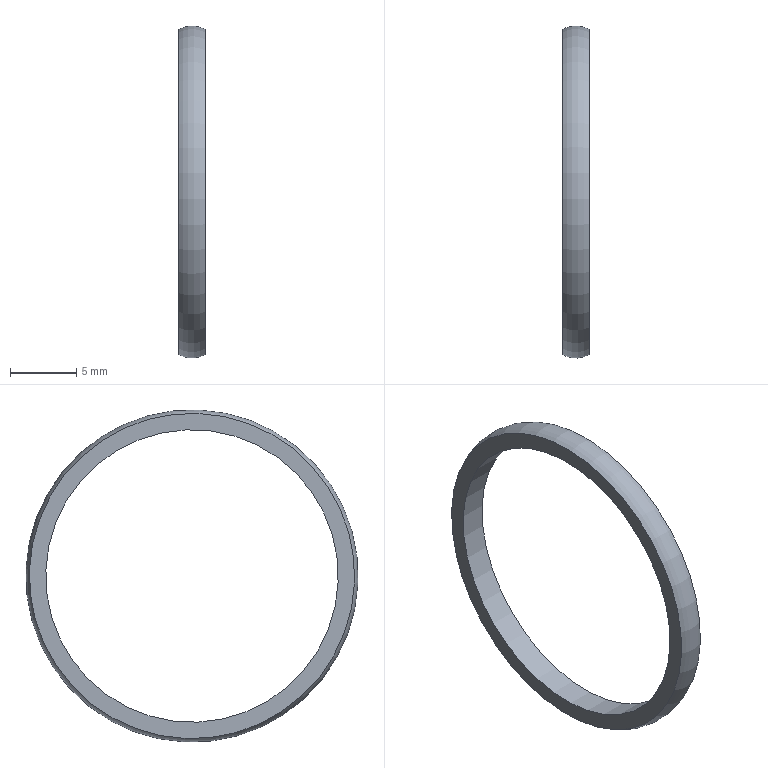Component | NX | PISTON_RING_2 | 1 solid | 4 faces | box 2 x 25 x 25 mm | volume 208 mm3 | plane 2 | torus 1 | cylinder 1 | commonest cylinder face diameters 22 x1
STEP:
#1=CARTESIAN_POINT('',(0.,0.,0.));
#2=DIRECTION('',(0.,0.,1.));
#3=DIRECTION('',(1.,0.,0.));
#4=AXIS2_PLACEMENT_3D('',#1,#2,#3);
#5=CARTESIAN_POINT('',(415.974,77.279,110.474));
#6=VERTEX_POINT('',#5);
#7=CARTESIAN_POINT('',(415.974,89.5,111.));
#8=DIRECTION('',(-1.,0.,0.));
#9=DIRECTION('',(0.,-0.9991,-0.04303));
#10=AXIS2_PLACEMENT_3D('',#7,#8,#9);
#11=CIRCLE('',#10,12.232);
#12=CARTESIAN_POINT('',(415.974,89.973,100.01));
#13=DIRECTION('',(-1.,0.,0.));
#14=DIRECTION('',(0.,-0.9991,-0.04303));
#15=AXIS2_PLACEMENT_3D('',#12,#13,#14);
#16=PLANE('',#15);
#17=CARTESIAN_POINT('',(0.,11.));
#18=DIRECTION('',(1.,-0.));
#19=AXIS2_PLACEMENT_2D('',#17,#18);
#20=CIRCLE('',#19,12.232);
#21=(GEOMETRIC_REPRESENTATION_CONTEXT(2)PARAMETRIC_REPRESENTATION_CONTEXT()REPRESENTATION_CONTEXT('',''));
#22=DEFINITIONAL_REPRESENTATION('',(#20),#21);
#23=PCURVE('',#16,#22);
#24=CARTESIAN_POINT('',(416.974,89.5,111.));
#25=DIRECTION('',(-1.,0.,0.));
#26=DIRECTION('',(0.,-0.9991,-0.04303));
#27=AXIS2_PLACEMENT_3D('',#24,#25,#26);
#28=TOROIDAL_SURFACE('',#27,10.5,2.);
#29=CARTESIAN_POINT('',(0.,6.807));
#30=DIRECTION('',(1.,0.));
#31=VECTOR('',#30,1.);
#32=LINE('',#29,#31);
#33=(GEOMETRIC_REPRESENTATION_CONTEXT(2)PARAMETRIC_REPRESENTATION_CONTEXT()REPRESENTATION_CONTEXT('',''));
#34=DEFINITIONAL_REPRESENTATION('',(#32),#33);
#35=PCURVE('',#28,#34);
#36=SURFACE_CURVE('',#11,(#23,#35),.PCURVE_S1.);
#37=EDGE_CURVE('',#6,#6,#36,.T.);
#38=ORIENTED_EDGE('',*,*,#37,.T.);
#39=EDGE_LOOP('',(#38));
#40=FACE_BOUND('',#39,.T.);
#41=CARTESIAN_POINT('',(415.974,78.51,110.527));
#42=VERTEX_POINT('',#41);
#43=CARTESIAN_POINT('',(415.974,89.5,111.));
#44=DIRECTION('',(-1.,0.,0.));
#45=DIRECTION('',(0.,-0.9991,-0.04303));
#46=AXIS2_PLACEMENT_3D('',#43,#44,#45);
#47=CIRCLE('',#46,11.);
#48=CARTESIAN_POINT('',(0.,11.));
#49=DIRECTION('',(1.,-0.));
#50=AXIS2_PLACEMENT_2D('',#48,#49);
#51=CIRCLE('',#50,11.);
#52=(GEOMETRIC_REPRESENTATION_CONTEXT(2)PARAMETRIC_REPRESENTATION_CONTEXT()REPRESENTATION_CONTEXT('',''));
#53=DEFINITIONAL_REPRESENTATION('',(#51),#52);
#54=PCURVE('',#16,#53);
#55=CARTESIAN_POINT('',(415.974,89.5,111.));
#56=DIRECTION('',(-1.,0.,0.));
#57=DIRECTION('',(0.,-0.9991,-0.04303));
#58=AXIS2_PLACEMENT_3D('',#55,#56,#57);
#59=CYLINDRICAL_SURFACE('',#58,11.);
#60=CARTESIAN_POINT('',(0.,0.));
#61=DIRECTION('',(1.,0.));
#62=VECTOR('',#61,1.);
#63=LINE('',#60,#62);
#64=(GEOMETRIC_REPRESENTATION_CONTEXT(2)PARAMETRIC_REPRESENTATION_CONTEXT()REPRESENTATION_CONTEXT('',''));
#65=DEFINITIONAL_REPRESENTATION('',(#63),#64);
#66=PCURVE('',#59,#65);
#67=SURFACE_CURVE('',#47,(#54,#66),.PCURVE_S1.);
#68=EDGE_CURVE('',#42,#42,#67,.T.);
#69=ORIENTED_EDGE('',*,*,#68,.F.);
#70=EDGE_LOOP('',(#69));
#71=FACE_BOUND('',#70,.T.);
#72=ADVANCED_FACE('',(#40,#71),#16,.T.);
#73=CARTESIAN_POINT('',(417.974,77.279,110.474));
#74=VERTEX_POINT('',#73);
#75=CARTESIAN_POINT('',(417.974,89.5,111.));
#76=DIRECTION('',(-1.,0.,0.));
#77=DIRECTION('',(0.,-0.9991,-0.04303));
#78=AXIS2_PLACEMENT_3D('',#75,#76,#77);
#79=CIRCLE('',#78,12.232);
#80=CARTESIAN_POINT('',(0.,5.76));
#81=DIRECTION('',(1.,0.));
#82=VECTOR('',#81,1.);
#83=LINE('',#80,#82);
#84=(GEOMETRIC_REPRESENTATION_CONTEXT(2)PARAMETRIC_REPRESENTATION_CONTEXT()REPRESENTATION_CONTEXT('',''));
#85=DEFINITIONAL_REPRESENTATION('',(#83),#84);
#86=PCURVE('',#28,#85);
#87=CARTESIAN_POINT('',(417.974,90.026,98.779));
#88=DIRECTION('',(1.,0.,0.));
#89=DIRECTION('',(0.,0.9991,0.04303));
#90=AXIS2_PLACEMENT_3D('',#87,#88,#89);
#91=PLANE('',#90);
#92=CARTESIAN_POINT('',(-12.232,12.232));
#93=CARTESIAN_POINT('',(-12.232,33.419));
#94=CARTESIAN_POINT('',(6.116,22.825));
#95=CARTESIAN_POINT('',(24.464,12.232));
#96=CARTESIAN_POINT('',(6.116,1.639));
#97=CARTESIAN_POINT('',(-12.232,-8.954));
#98=CARTESIAN_POINT('',(-12.232,12.232));
#99=(BOUNDED_CURVE()B_SPLINE_CURVE(2,(#92,#93,#94,#95,#96,#97,#98),.UNSPECIFIED.,.T.,.F.)B_SPLINE_CURVE_WITH_KNOTS((1,2,2,2,2,1),(-2.094,0.,2.094,4.189,6.283,8.378),.UNSPECIFIED.)CURVE()GEOMETRIC_REPRESENTATION_ITEM()RATIONAL_B_SPLINE_CURVE((1.,0.5,1.,0.5,1.,0.5,1.))REPRESENTATION_ITEM(''));
#100=(GEOMETRIC_REPRESENTATION_CONTEXT(2)PARAMETRIC_REPRESENTATION_CONTEXT()REPRESENTATION_CONTEXT('',''));
#101=DEFINITIONAL_REPRESENTATION('',(#99),#100);
#102=PCURVE('',#91,#101);
#103=SURFACE_CURVE('',#79,(#86,#102),.PCURVE_S1.);
#104=EDGE_CURVE('',#74,#74,#103,.T.);
#105=ORIENTED_EDGE('',*,*,#104,.T.);
#106=CARTESIAN_POINT('',(417.974,77.279,110.474));
#107=CARTESIAN_POINT('',(417.611,77.07,110.465));
#108=CARTESIAN_POINT('',(417.193,76.956,110.46));
#109=CARTESIAN_POINT('',(416.754,76.956,110.46));
#110=CARTESIAN_POINT('',(416.336,77.07,110.465));
#111=CARTESIAN_POINT('',(415.974,77.279,110.474));
#112=B_SPLINE_CURVE_WITH_KNOTS('',5,(#106,#107,#108,#109,#110,#111),.UNSPECIFIED.,.F.,.F.,(6,6),(5.76,6.807),.PIECEWISE_BEZIER_KNOTS.);
#113=CARTESIAN_POINT('',(6.283,0.));
#114=DIRECTION('',(0.,1.));
#115=VECTOR('',#114,1.);
#116=LINE('',#113,#115);
#117=(GEOMETRIC_REPRESENTATION_CONTEXT(2)PARAMETRIC_REPRESENTATION_CONTEXT()REPRESENTATION_CONTEXT('',''));
#118=DEFINITIONAL_REPRESENTATION('',(#116),#117);
#119=PCURVE('',#28,#118);
#120=CARTESIAN_POINT('',(0.,0.));
#121=DIRECTION('',(0.,1.));
#122=VECTOR('',#121,1.);
#123=LINE('',#120,#122);
#124=(GEOMETRIC_REPRESENTATION_CONTEXT(2)PARAMETRIC_REPRESENTATION_CONTEXT()REPRESENTATION_CONTEXT('',''));
#125=DEFINITIONAL_REPRESENTATION('',(#123),#124);
#126=PCURVE('',#28,#125);
#127=SEAM_CURVE('',#112,(#119,#126),.PCURVE_S1.);
#128=EDGE_CURVE('',#74,#6,#127,.T.);
#129=ORIENTED_EDGE('',*,*,#128,.T.);
#130=ORIENTED_EDGE('',*,*,#37,.F.);
#131=ORIENTED_EDGE('',*,*,#128,.F.);
#132=EDGE_LOOP('',(#105,#129,#130,#131));
#133=FACE_BOUND('',#132,.T.);
#134=ADVANCED_FACE('',(#133),#28,.T.);
#135=CARTESIAN_POINT('',(417.974,78.51,110.527));
#136=VERTEX_POINT('',#135);
#137=CARTESIAN_POINT('',(417.974,89.5,111.));
#138=DIRECTION('',(-1.,0.,0.));
#139=DIRECTION('',(0.,-0.9991,-0.04303));
#140=AXIS2_PLACEMENT_3D('',#137,#138,#139);
#141=CIRCLE('',#140,11.);
#142=CARTESIAN_POINT('',(-11.,12.232));
#143=CARTESIAN_POINT('',(-11.,31.285));
#144=CARTESIAN_POINT('',(5.5,21.758));
#145=CARTESIAN_POINT('',(22.,12.232));
#146=CARTESIAN_POINT('',(5.5,2.706));
#147=CARTESIAN_POINT('',(-11.,-6.821));
#148=CARTESIAN_POINT('',(-11.,12.232));
#149=(BOUNDED_CURVE()B_SPLINE_CURVE(2,(#142,#143,#144,#145,#146,#147,#148),.UNSPECIFIED.,.T.,.F.)B_SPLINE_CURVE_WITH_KNOTS((1,2,2,2,2,1),(-2.094,0.,2.094,4.189,6.283,8.378),.UNSPECIFIED.)CURVE()GEOMETRIC_REPRESENTATION_ITEM()RATIONAL_B_SPLINE_CURVE((1.,0.5,1.,0.5,1.,0.5,1.))REPRESENTATION_ITEM(''));
#150=(GEOMETRIC_REPRESENTATION_CONTEXT(2)PARAMETRIC_REPRESENTATION_CONTEXT()REPRESENTATION_CONTEXT('',''));
#151=DEFINITIONAL_REPRESENTATION('',(#149),#150);
#152=PCURVE('',#91,#151);
#153=CARTESIAN_POINT('',(0.,-2.));
#154=DIRECTION('',(1.,0.));
#155=VECTOR('',#154,1.);
#156=LINE('',#153,#155);
#157=(GEOMETRIC_REPRESENTATION_CONTEXT(2)PARAMETRIC_REPRESENTATION_CONTEXT()REPRESENTATION_CONTEXT('',''));
#158=DEFINITIONAL_REPRESENTATION('',(#156),#157);
#159=PCURVE('',#59,#158);
#160=SURFACE_CURVE('',#141,(#152,#159),.PCURVE_S1.);
#161=EDGE_CURVE('',#136,#136,#160,.T.);
#162=ORIENTED_EDGE('',*,*,#161,.T.);
#163=EDGE_LOOP('',(#162));
#164=FACE_BOUND('',#163,.T.);
#165=ORIENTED_EDGE('',*,*,#104,.F.);
#166=EDGE_LOOP('',(#165));
#167=FACE_BOUND('',#166,.T.);
#168=ADVANCED_FACE('',(#164,#167),#91,.T.);
#169=ORIENTED_EDGE('',*,*,#68,.F.);
#170=CARTESIAN_POINT('',(417.974,78.51,110.527));
#171=CARTESIAN_POINT('',(415.974,78.51,110.527));
#172=B_SPLINE_CURVE_WITH_KNOTS('',1,(#170,#171),.UNSPECIFIED.,.F.,.F.,(2,2),(-2.,0.),.PIECEWISE_BEZIER_KNOTS.);
#173=CARTESIAN_POINT('',(0.,0.));
#174=DIRECTION('',(0.,1.));
#175=VECTOR('',#174,1.);
#176=LINE('',#173,#175);
#177=(GEOMETRIC_REPRESENTATION_CONTEXT(2)PARAMETRIC_REPRESENTATION_CONTEXT()REPRESENTATION_CONTEXT('',''));
#178=DEFINITIONAL_REPRESENTATION('',(#176),#177);
#179=PCURVE('',#59,#178);
#180=CARTESIAN_POINT('',(6.283,0.));
#181=DIRECTION('',(0.,1.));
#182=VECTOR('',#181,1.);
#183=LINE('',#180,#182);
#184=(GEOMETRIC_REPRESENTATION_CONTEXT(2)PARAMETRIC_REPRESENTATION_CONTEXT()REPRESENTATION_CONTEXT('',''));
#185=DEFINITIONAL_REPRESENTATION('',(#183),#184);
#186=PCURVE('',#59,#185);
#187=SEAM_CURVE('',#172,(#179,#186),.PCURVE_S1.);
#188=EDGE_CURVE('',#136,#42,#187,.T.);
#189=ORIENTED_EDGE('',*,*,#188,.F.);
#190=ORIENTED_EDGE('',*,*,#161,.T.);
#191=ORIENTED_EDGE('',*,*,#188,.T.);
#192=EDGE_LOOP('',(#169,#189,#190,#191));
#193=FACE_BOUND('',#192,.F.);
#194=ADVANCED_FACE('',(#193),#59,.F.);
#195=CLOSED_SHELL('',(#72,#134,#168,#194));
#196=MANIFOLD_SOLID_BREP('',#195);
#197=(LENGTH_UNIT()NAMED_UNIT(*)SI_UNIT(.MILLI.,.METRE.));
#198=UNCERTAINTY_MEASURE_WITH_UNIT(LENGTH_MEASURE(0.00001),#197,'','');
#199=(NAMED_UNIT(*)PLANE_ANGLE_UNIT()SI_UNIT($,.RADIAN.));
#200=(NAMED_UNIT(*)SI_UNIT($,.STERADIAN.)SOLID_ANGLE_UNIT());
#201=(GEOMETRIC_REPRESENTATION_CONTEXT(3)GLOBAL_UNCERTAINTY_ASSIGNED_CONTEXT((#198))GLOBAL_UNIT_ASSIGNED_CONTEXT((#197,#199,#200))REPRESENTATION_CONTEXT('',''));
#202=ADVANCED_BREP_SHAPE_REPRESENTATION('',(#4,#196),#201);